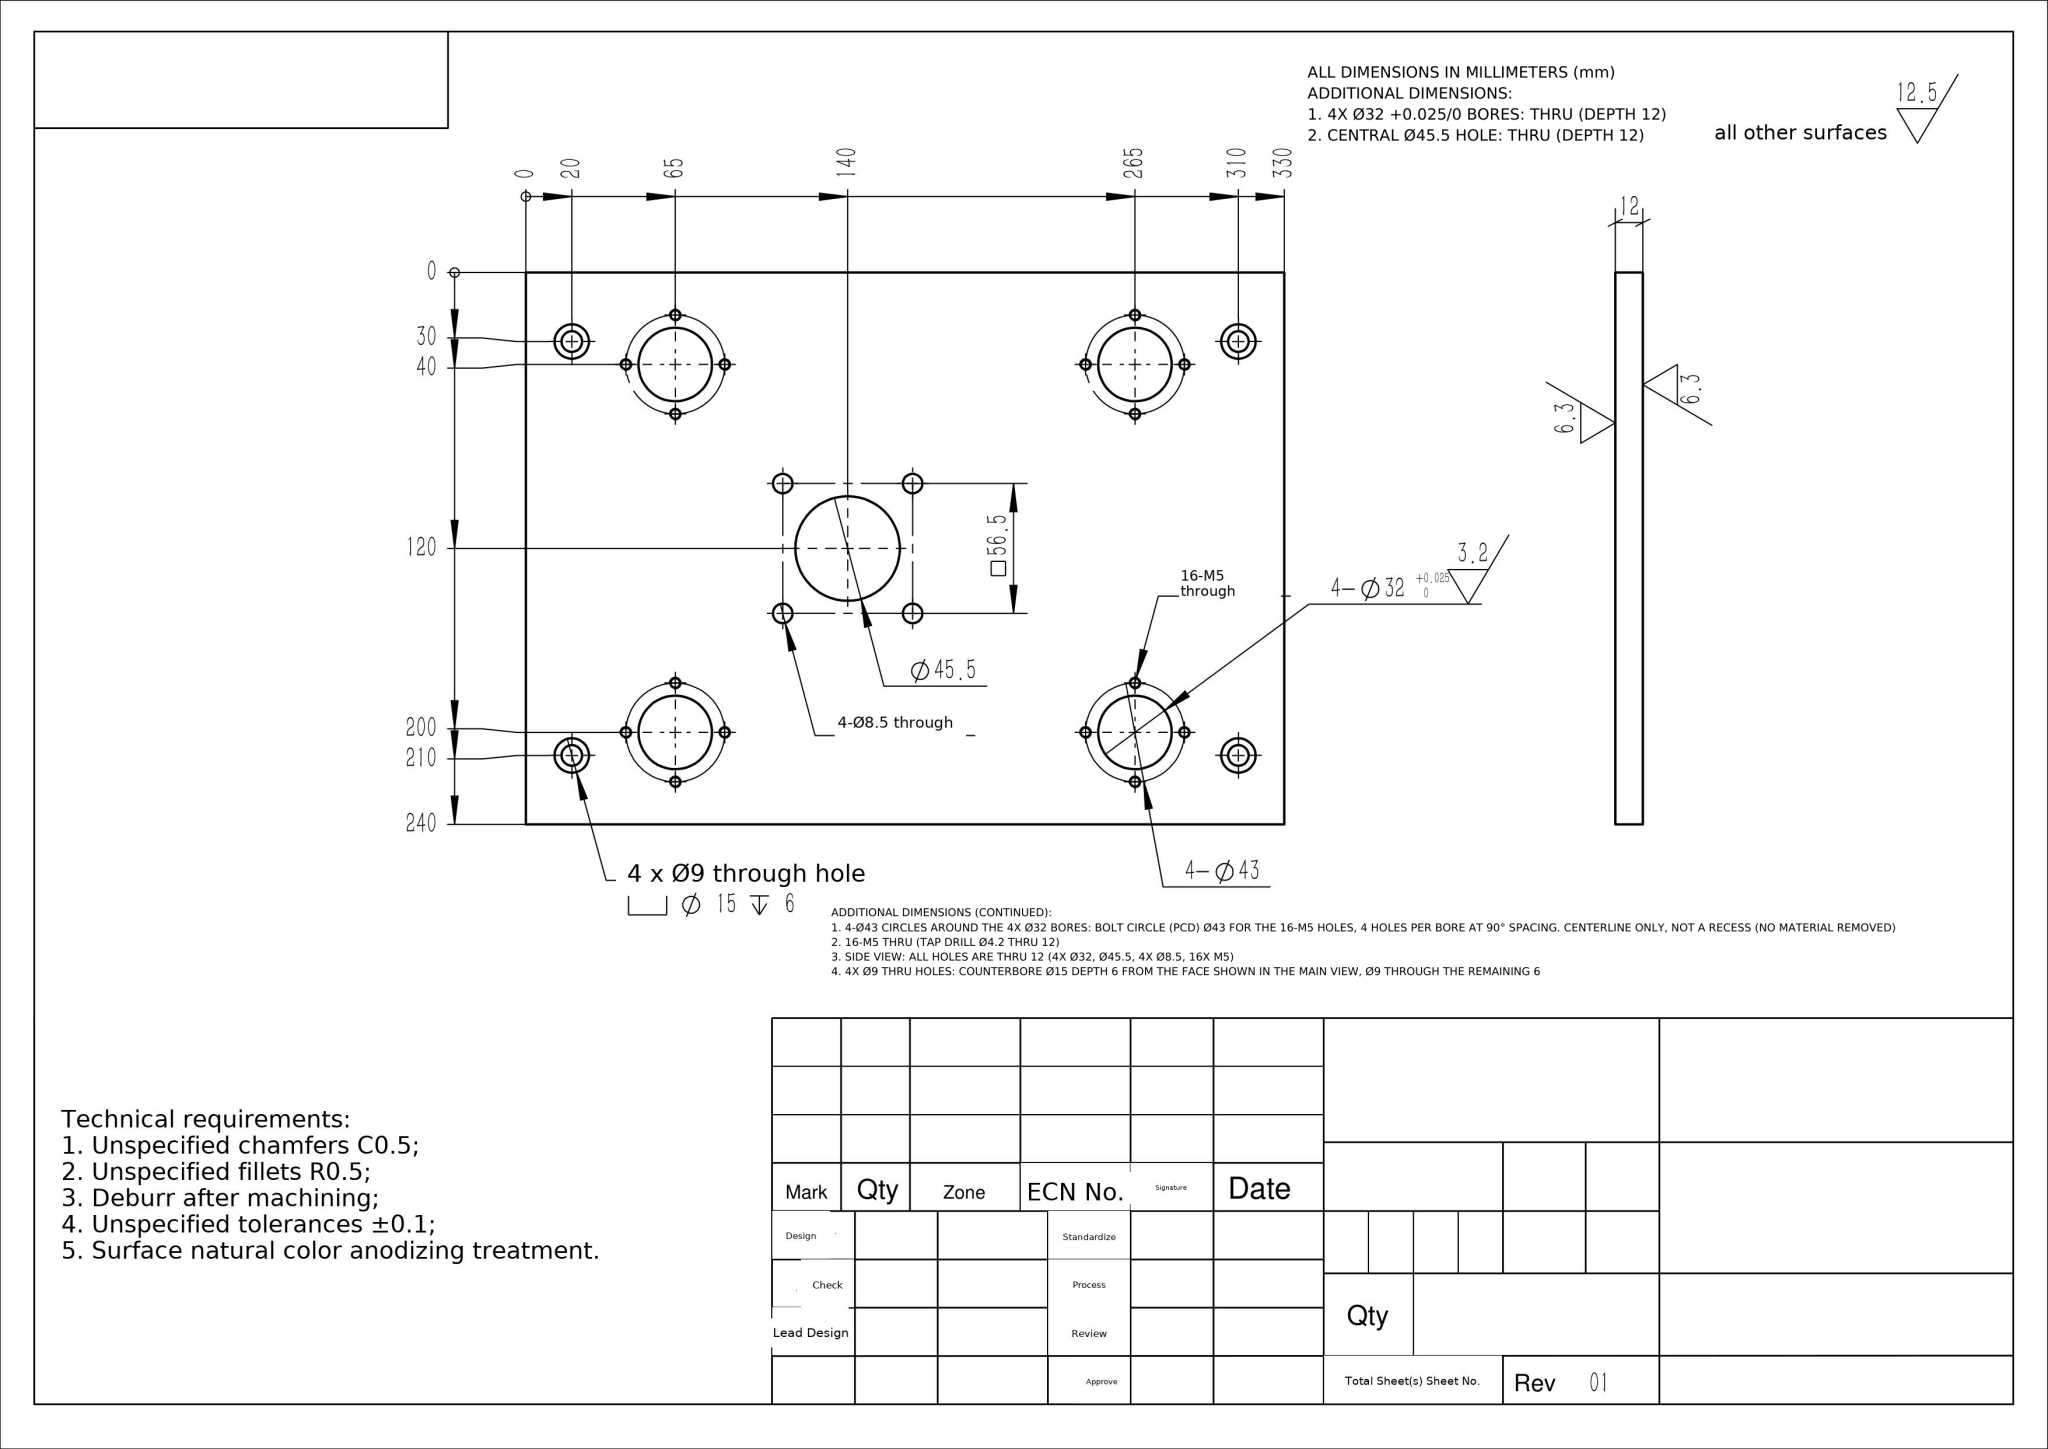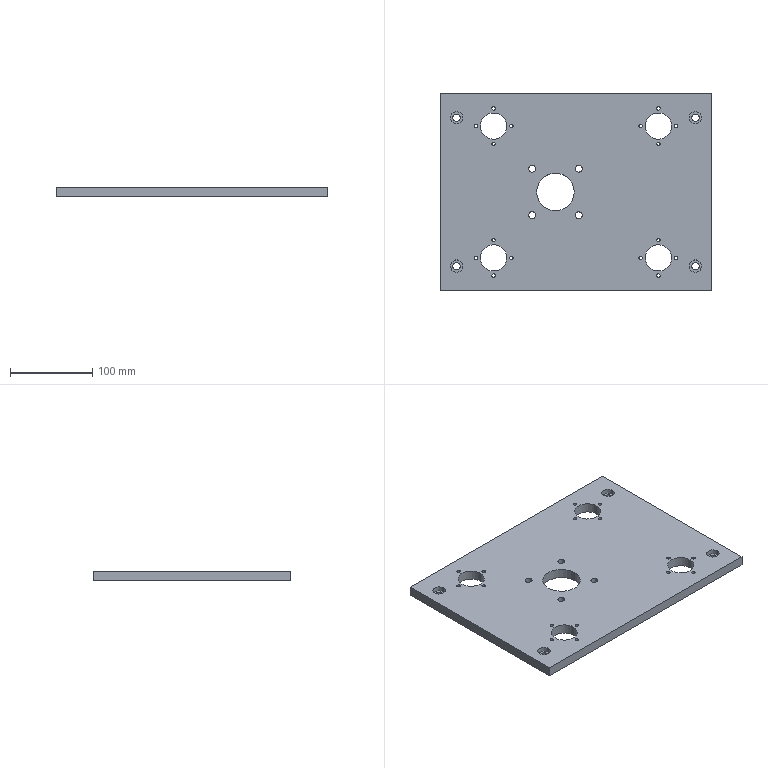Part | NX | mm | 1 solid | 76 faces | box 330 x 240 x 12 mm | volume 881133 mm3 | cylinder 66 | plane 10 | commonest cylinder face diameters 4.2 x32 15 x8 9 x8 32 x8 8.5 x8 45.5 x2